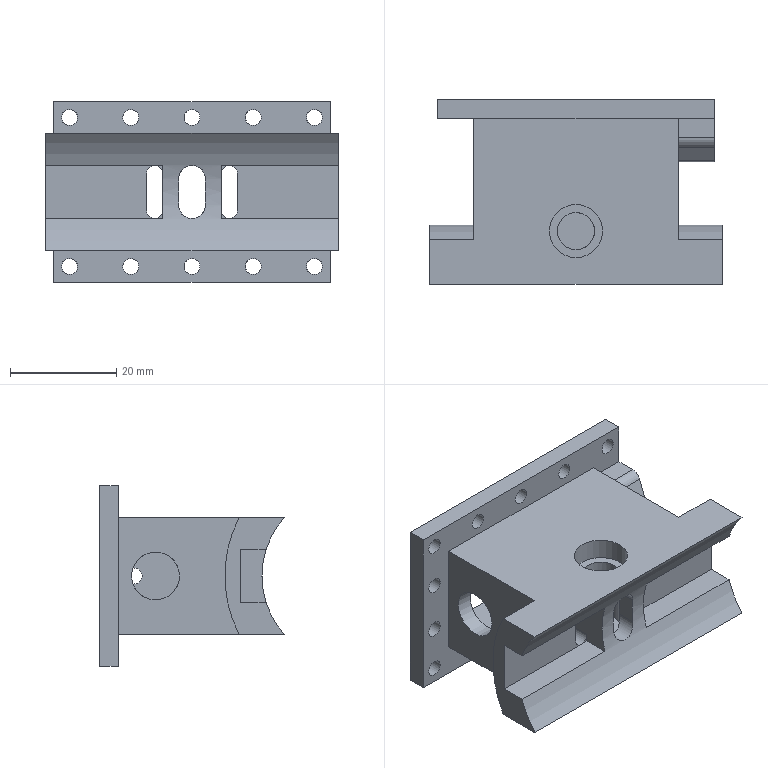Component | NX | EXT_CYLINDER_BODY | 1 solid | 81 faces | volume 20160 mm3 | plane 46 | cylinder 35 | commonest cylinder face diameters 3 x19 5 x4 47 x2 7 x2 9 x2 4 x2 2.5 x2 33 x1